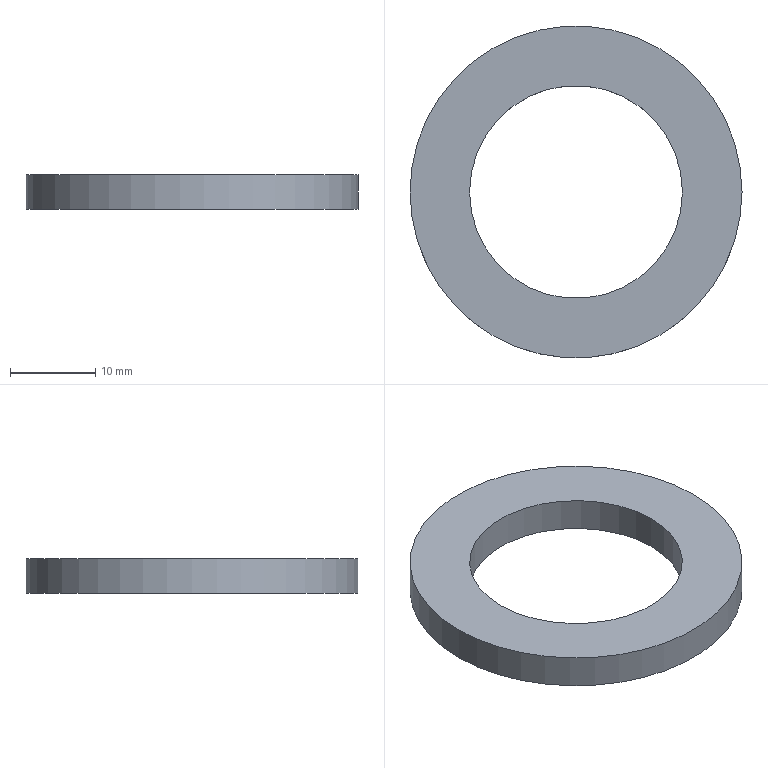Component | NX | GB-T848-2002_M24 | 1 solid | 4 faces | box 39 x 39 x 4 mm | volume 2815 mm3 | cylinder 2 | plane 2 | commonest cylinder face diameters 39 x1 25 x1
STEP:
#1=CARTESIAN_POINT('',(0.,0.,0.));
#2=DIRECTION('',(0.,0.,1.));
#3=DIRECTION('',(1.,0.,0.));
#4=AXIS2_PLACEMENT_3D('',#1,#2,#3);
#5=CARTESIAN_POINT('',(189.5,-80.,294.));
#6=VERTEX_POINT('',#5);
#7=CARTESIAN_POINT('',(170.,-80.,294.));
#8=DIRECTION('',(0.,0.,1.));
#9=DIRECTION('',(1.,0.,0.));
#10=AXIS2_PLACEMENT_3D('',#7,#8,#9);
#11=CIRCLE('',#10,19.5);
#12=CARTESIAN_POINT('',(170.,-80.,294.));
#13=DIRECTION('',(0.,0.,-1.));
#14=DIRECTION('',(-1.,0.,0.));
#15=AXIS2_PLACEMENT_3D('',#12,#13,#14);
#16=CYLINDRICAL_SURFACE('',#15,19.5);
#17=CARTESIAN_POINT('',(9.425,0.));
#18=DIRECTION('',(-1.,0.));
#19=VECTOR('',#18,1.);
#20=LINE('',#17,#19);
#21=(GEOMETRIC_REPRESENTATION_CONTEXT(2)PARAMETRIC_REPRESENTATION_CONTEXT()REPRESENTATION_CONTEXT('',''));
#22=DEFINITIONAL_REPRESENTATION('',(#20),#21);
#23=PCURVE('',#16,#22);
#24=CARTESIAN_POINT('',(170.,-80.,294.));
#25=DIRECTION('',(0.,0.,1.));
#26=DIRECTION('',(1.,0.,0.));
#27=AXIS2_PLACEMENT_3D('',#24,#25,#26);
#28=PLANE('',#27);
#29=CARTESIAN_POINT('',(0.,0.));
#30=DIRECTION('',(1.,0.));
#31=AXIS2_PLACEMENT_2D('',#29,#30);
#32=CIRCLE('',#31,19.5);
#33=(GEOMETRIC_REPRESENTATION_CONTEXT(2)PARAMETRIC_REPRESENTATION_CONTEXT()REPRESENTATION_CONTEXT('',''));
#34=DEFINITIONAL_REPRESENTATION('',(#32),#33);
#35=PCURVE('',#28,#34);
#36=SURFACE_CURVE('',#11,(#23,#35),.PCURVE_S1.);
#37=EDGE_CURVE('',#6,#6,#36,.T.);
#38=ORIENTED_EDGE('',*,*,#37,.F.);
#39=CARTESIAN_POINT('',(189.5,-80.,290.));
#40=VERTEX_POINT('',#39);
#41=CARTESIAN_POINT('',(189.5,-80.,294.));
#42=CARTESIAN_POINT('',(189.5,-80.,290.));
#43=B_SPLINE_CURVE_WITH_KNOTS('',1,(#41,#42),.UNSPECIFIED.,.F.,.F.,(2,2),(0.,4.),.PIECEWISE_BEZIER_KNOTS.);
#44=CARTESIAN_POINT('',(9.425,0.));
#45=DIRECTION('',(0.,1.));
#46=VECTOR('',#45,1.);
#47=LINE('',#44,#46);
#48=(GEOMETRIC_REPRESENTATION_CONTEXT(2)PARAMETRIC_REPRESENTATION_CONTEXT()REPRESENTATION_CONTEXT('',''));
#49=DEFINITIONAL_REPRESENTATION('',(#47),#48);
#50=PCURVE('',#16,#49);
#51=CARTESIAN_POINT('',(3.142,0.));
#52=DIRECTION('',(0.,1.));
#53=VECTOR('',#52,1.);
#54=LINE('',#51,#53);
#55=(GEOMETRIC_REPRESENTATION_CONTEXT(2)PARAMETRIC_REPRESENTATION_CONTEXT()REPRESENTATION_CONTEXT('',''));
#56=DEFINITIONAL_REPRESENTATION('',(#54),#55);
#57=PCURVE('',#16,#56);
#58=SEAM_CURVE('',#43,(#50,#57),.PCURVE_S1.);
#59=EDGE_CURVE('',#6,#40,#58,.T.);
#60=ORIENTED_EDGE('',*,*,#59,.T.);
#61=CARTESIAN_POINT('',(170.,-80.,290.));
#62=DIRECTION('',(0.,0.,1.));
#63=DIRECTION('',(1.,0.,0.));
#64=AXIS2_PLACEMENT_3D('',#61,#62,#63);
#65=CIRCLE('',#64,19.5);
#66=CARTESIAN_POINT('',(9.425,4.));
#67=DIRECTION('',(-1.,0.));
#68=VECTOR('',#67,1.);
#69=LINE('',#66,#68);
#70=(GEOMETRIC_REPRESENTATION_CONTEXT(2)PARAMETRIC_REPRESENTATION_CONTEXT()REPRESENTATION_CONTEXT('',''));
#71=DEFINITIONAL_REPRESENTATION('',(#69),#70);
#72=PCURVE('',#16,#71);
#73=CARTESIAN_POINT('',(170.,-80.,290.));
#74=DIRECTION('',(0.,0.,1.));
#75=DIRECTION('',(1.,0.,0.));
#76=AXIS2_PLACEMENT_3D('',#73,#74,#75);
#77=PLANE('',#76);
#78=CARTESIAN_POINT('',(0.,0.));
#79=DIRECTION('',(1.,0.));
#80=AXIS2_PLACEMENT_2D('',#78,#79);
#81=CIRCLE('',#80,19.5);
#82=(GEOMETRIC_REPRESENTATION_CONTEXT(2)PARAMETRIC_REPRESENTATION_CONTEXT()REPRESENTATION_CONTEXT('',''));
#83=DEFINITIONAL_REPRESENTATION('',(#81),#82);
#84=PCURVE('',#77,#83);
#85=SURFACE_CURVE('',#65,(#72,#84),.PCURVE_S1.);
#86=EDGE_CURVE('',#40,#40,#85,.T.);
#87=ORIENTED_EDGE('',*,*,#86,.T.);
#88=ORIENTED_EDGE('',*,*,#59,.F.);
#89=EDGE_LOOP('',(#38,#60,#87,#88));
#90=FACE_BOUND('',#89,.T.);
#91=ADVANCED_FACE('',(#90),#16,.T.);
#92=CARTESIAN_POINT('',(182.5,-80.,294.));
#93=VERTEX_POINT('',#92);
#94=CARTESIAN_POINT('',(170.,-80.,294.));
#95=DIRECTION('',(0.,0.,1.));
#96=DIRECTION('',(1.,0.,0.));
#97=AXIS2_PLACEMENT_3D('',#94,#95,#96);
#98=CIRCLE('',#97,12.5);
#99=CARTESIAN_POINT('',(170.,-80.,294.));
#100=DIRECTION('',(0.,0.,-1.));
#101=DIRECTION('',(-1.,0.,0.));
#102=AXIS2_PLACEMENT_3D('',#99,#100,#101);
#103=CYLINDRICAL_SURFACE('',#102,12.5);
#104=CARTESIAN_POINT('',(9.425,0.));
#105=DIRECTION('',(-1.,0.));
#106=VECTOR('',#105,1.);
#107=LINE('',#104,#106);
#108=(GEOMETRIC_REPRESENTATION_CONTEXT(2)PARAMETRIC_REPRESENTATION_CONTEXT()REPRESENTATION_CONTEXT('',''));
#109=DEFINITIONAL_REPRESENTATION('',(#107),#108);
#110=PCURVE('',#103,#109);
#111=CARTESIAN_POINT('',(0.,0.));
#112=DIRECTION('',(1.,0.));
#113=AXIS2_PLACEMENT_2D('',#111,#112);
#114=CIRCLE('',#113,12.5);
#115=(GEOMETRIC_REPRESENTATION_CONTEXT(2)PARAMETRIC_REPRESENTATION_CONTEXT()REPRESENTATION_CONTEXT('',''));
#116=DEFINITIONAL_REPRESENTATION('',(#114),#115);
#117=PCURVE('',#28,#116);
#118=SURFACE_CURVE('',#98,(#110,#117),.PCURVE_S1.);
#119=EDGE_CURVE('',#93,#93,#118,.T.);
#120=ORIENTED_EDGE('',*,*,#119,.F.);
#121=CARTESIAN_POINT('',(182.5,-80.,290.));
#122=VERTEX_POINT('',#121);
#123=CARTESIAN_POINT('',(182.5,-80.,294.));
#124=CARTESIAN_POINT('',(182.5,-80.,290.));
#125=B_SPLINE_CURVE_WITH_KNOTS('',1,(#123,#124),.UNSPECIFIED.,.F.,.F.,(2,2),(0.,4.),.PIECEWISE_BEZIER_KNOTS.);
#126=CARTESIAN_POINT('',(9.425,0.));
#127=DIRECTION('',(0.,1.));
#128=VECTOR('',#127,1.);
#129=LINE('',#126,#128);
#130=(GEOMETRIC_REPRESENTATION_CONTEXT(2)PARAMETRIC_REPRESENTATION_CONTEXT()REPRESENTATION_CONTEXT('',''));
#131=DEFINITIONAL_REPRESENTATION('',(#129),#130);
#132=PCURVE('',#103,#131);
#133=CARTESIAN_POINT('',(3.142,0.));
#134=DIRECTION('',(0.,1.));
#135=VECTOR('',#134,1.);
#136=LINE('',#133,#135);
#137=(GEOMETRIC_REPRESENTATION_CONTEXT(2)PARAMETRIC_REPRESENTATION_CONTEXT()REPRESENTATION_CONTEXT('',''));
#138=DEFINITIONAL_REPRESENTATION('',(#136),#137);
#139=PCURVE('',#103,#138);
#140=SEAM_CURVE('',#125,(#132,#139),.PCURVE_S1.);
#141=EDGE_CURVE('',#93,#122,#140,.T.);
#142=ORIENTED_EDGE('',*,*,#141,.T.);
#143=CARTESIAN_POINT('',(170.,-80.,290.));
#144=DIRECTION('',(0.,0.,1.));
#145=DIRECTION('',(1.,0.,0.));
#146=AXIS2_PLACEMENT_3D('',#143,#144,#145);
#147=CIRCLE('',#146,12.5);
#148=CARTESIAN_POINT('',(9.425,4.));
#149=DIRECTION('',(-1.,0.));
#150=VECTOR('',#149,1.);
#151=LINE('',#148,#150);
#152=(GEOMETRIC_REPRESENTATION_CONTEXT(2)PARAMETRIC_REPRESENTATION_CONTEXT()REPRESENTATION_CONTEXT('',''));
#153=DEFINITIONAL_REPRESENTATION('',(#151),#152);
#154=PCURVE('',#103,#153);
#155=CARTESIAN_POINT('',(0.,0.));
#156=DIRECTION('',(1.,0.));
#157=AXIS2_PLACEMENT_2D('',#155,#156);
#158=CIRCLE('',#157,12.5);
#159=(GEOMETRIC_REPRESENTATION_CONTEXT(2)PARAMETRIC_REPRESENTATION_CONTEXT()REPRESENTATION_CONTEXT('',''));
#160=DEFINITIONAL_REPRESENTATION('',(#158),#159);
#161=PCURVE('',#77,#160);
#162=SURFACE_CURVE('',#147,(#154,#161),.PCURVE_S1.);
#163=EDGE_CURVE('',#122,#122,#162,.T.);
#164=ORIENTED_EDGE('',*,*,#163,.T.);
#165=ORIENTED_EDGE('',*,*,#141,.F.);
#166=EDGE_LOOP('',(#120,#142,#164,#165));
#167=FACE_BOUND('',#166,.F.);
#168=ADVANCED_FACE('',(#167),#103,.F.);
#169=ORIENTED_EDGE('',*,*,#37,.T.);
#170=EDGE_LOOP('',(#169));
#171=FACE_BOUND('',#170,.T.);
#172=ORIENTED_EDGE('',*,*,#119,.F.);
#173=EDGE_LOOP('',(#172));
#174=FACE_BOUND('',#173,.T.);
#175=ADVANCED_FACE('',(#171,#174),#28,.T.);
#176=ORIENTED_EDGE('',*,*,#86,.F.);
#177=EDGE_LOOP('',(#176));
#178=FACE_BOUND('',#177,.T.);
#179=ORIENTED_EDGE('',*,*,#163,.T.);
#180=EDGE_LOOP('',(#179));
#181=FACE_BOUND('',#180,.T.);
#182=ADVANCED_FACE('',(#178,#181),#77,.F.);
#183=CLOSED_SHELL('',(#91,#168,#175,#182));
#184=MANIFOLD_SOLID_BREP('',#183);
#185=(LENGTH_UNIT()NAMED_UNIT(*)SI_UNIT(.MILLI.,.METRE.));
#186=UNCERTAINTY_MEASURE_WITH_UNIT(LENGTH_MEASURE(0.00001),#185,'','');
#187=(NAMED_UNIT(*)PLANE_ANGLE_UNIT()SI_UNIT($,.RADIAN.));
#188=(NAMED_UNIT(*)SI_UNIT($,.STERADIAN.)SOLID_ANGLE_UNIT());
#189=(GEOMETRIC_REPRESENTATION_CONTEXT(3)GLOBAL_UNCERTAINTY_ASSIGNED_CONTEXT((#186))GLOBAL_UNIT_ASSIGNED_CONTEXT((#185,#187,#188))REPRESENTATION_CONTEXT('',''));
#190=ADVANCED_BREP_SHAPE_REPRESENTATION('',(#4,#184),#189);